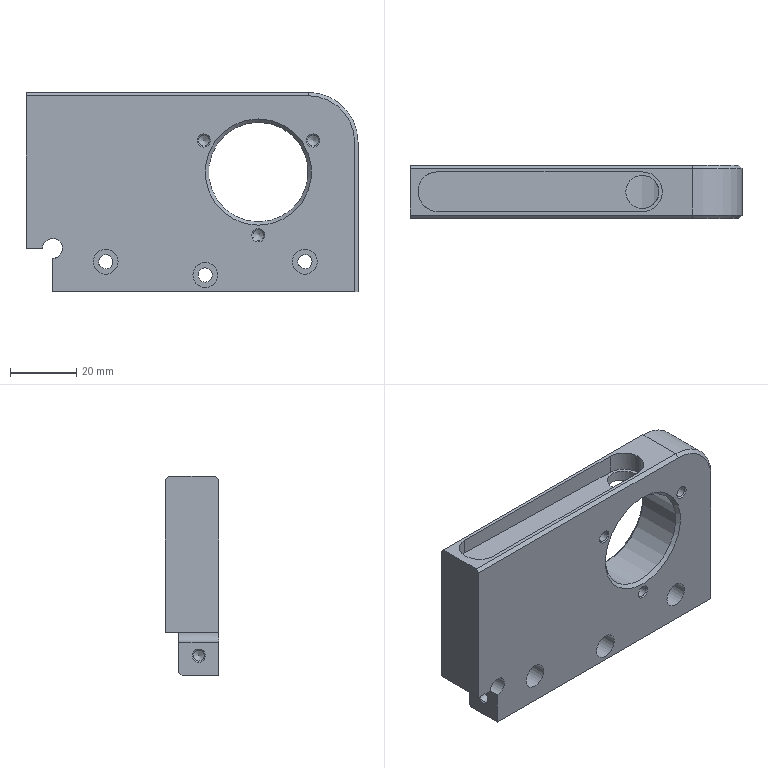Component | NX | LEFT_PLATE | 1 solid | 52 faces | volume 70522 mm3 | plane 22 | cylinder 18 | cone 12 | commonest cylinder face diameters 3.3 x4 12 x3 7.5 x3 4.3 x3 30 x2 6 x1 11 x1 10 x1